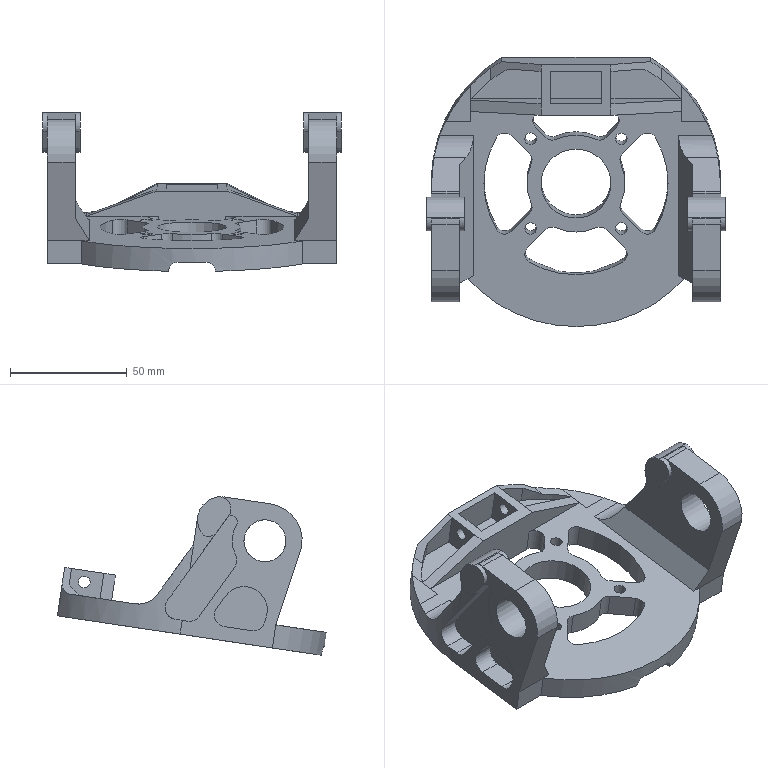Component | NX | ROTOR_BASE | 1 solid | 150 faces | volume 128746 mm3 | plane 79 | cylinder 71 | commonest cylinder face diameters 8 x18 10 x10 5 x8 20 x4 42 x4 8.063 x4 79 x3 124 x3